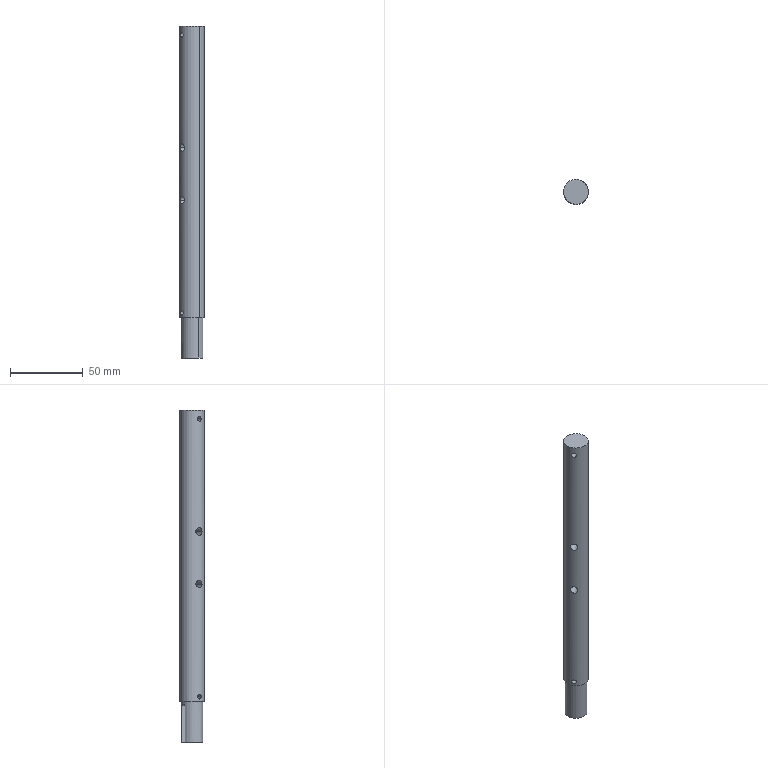Component | SolidWorks | XT-1-13-2-1 | 1 solid | 24 faces | volume 49077 mm3 | cylinder 14 | plane 6 | cone 4 | commonest cylinder face diameters 5.2 x4 3.3 x4 17 x2 15 x2 4 x2